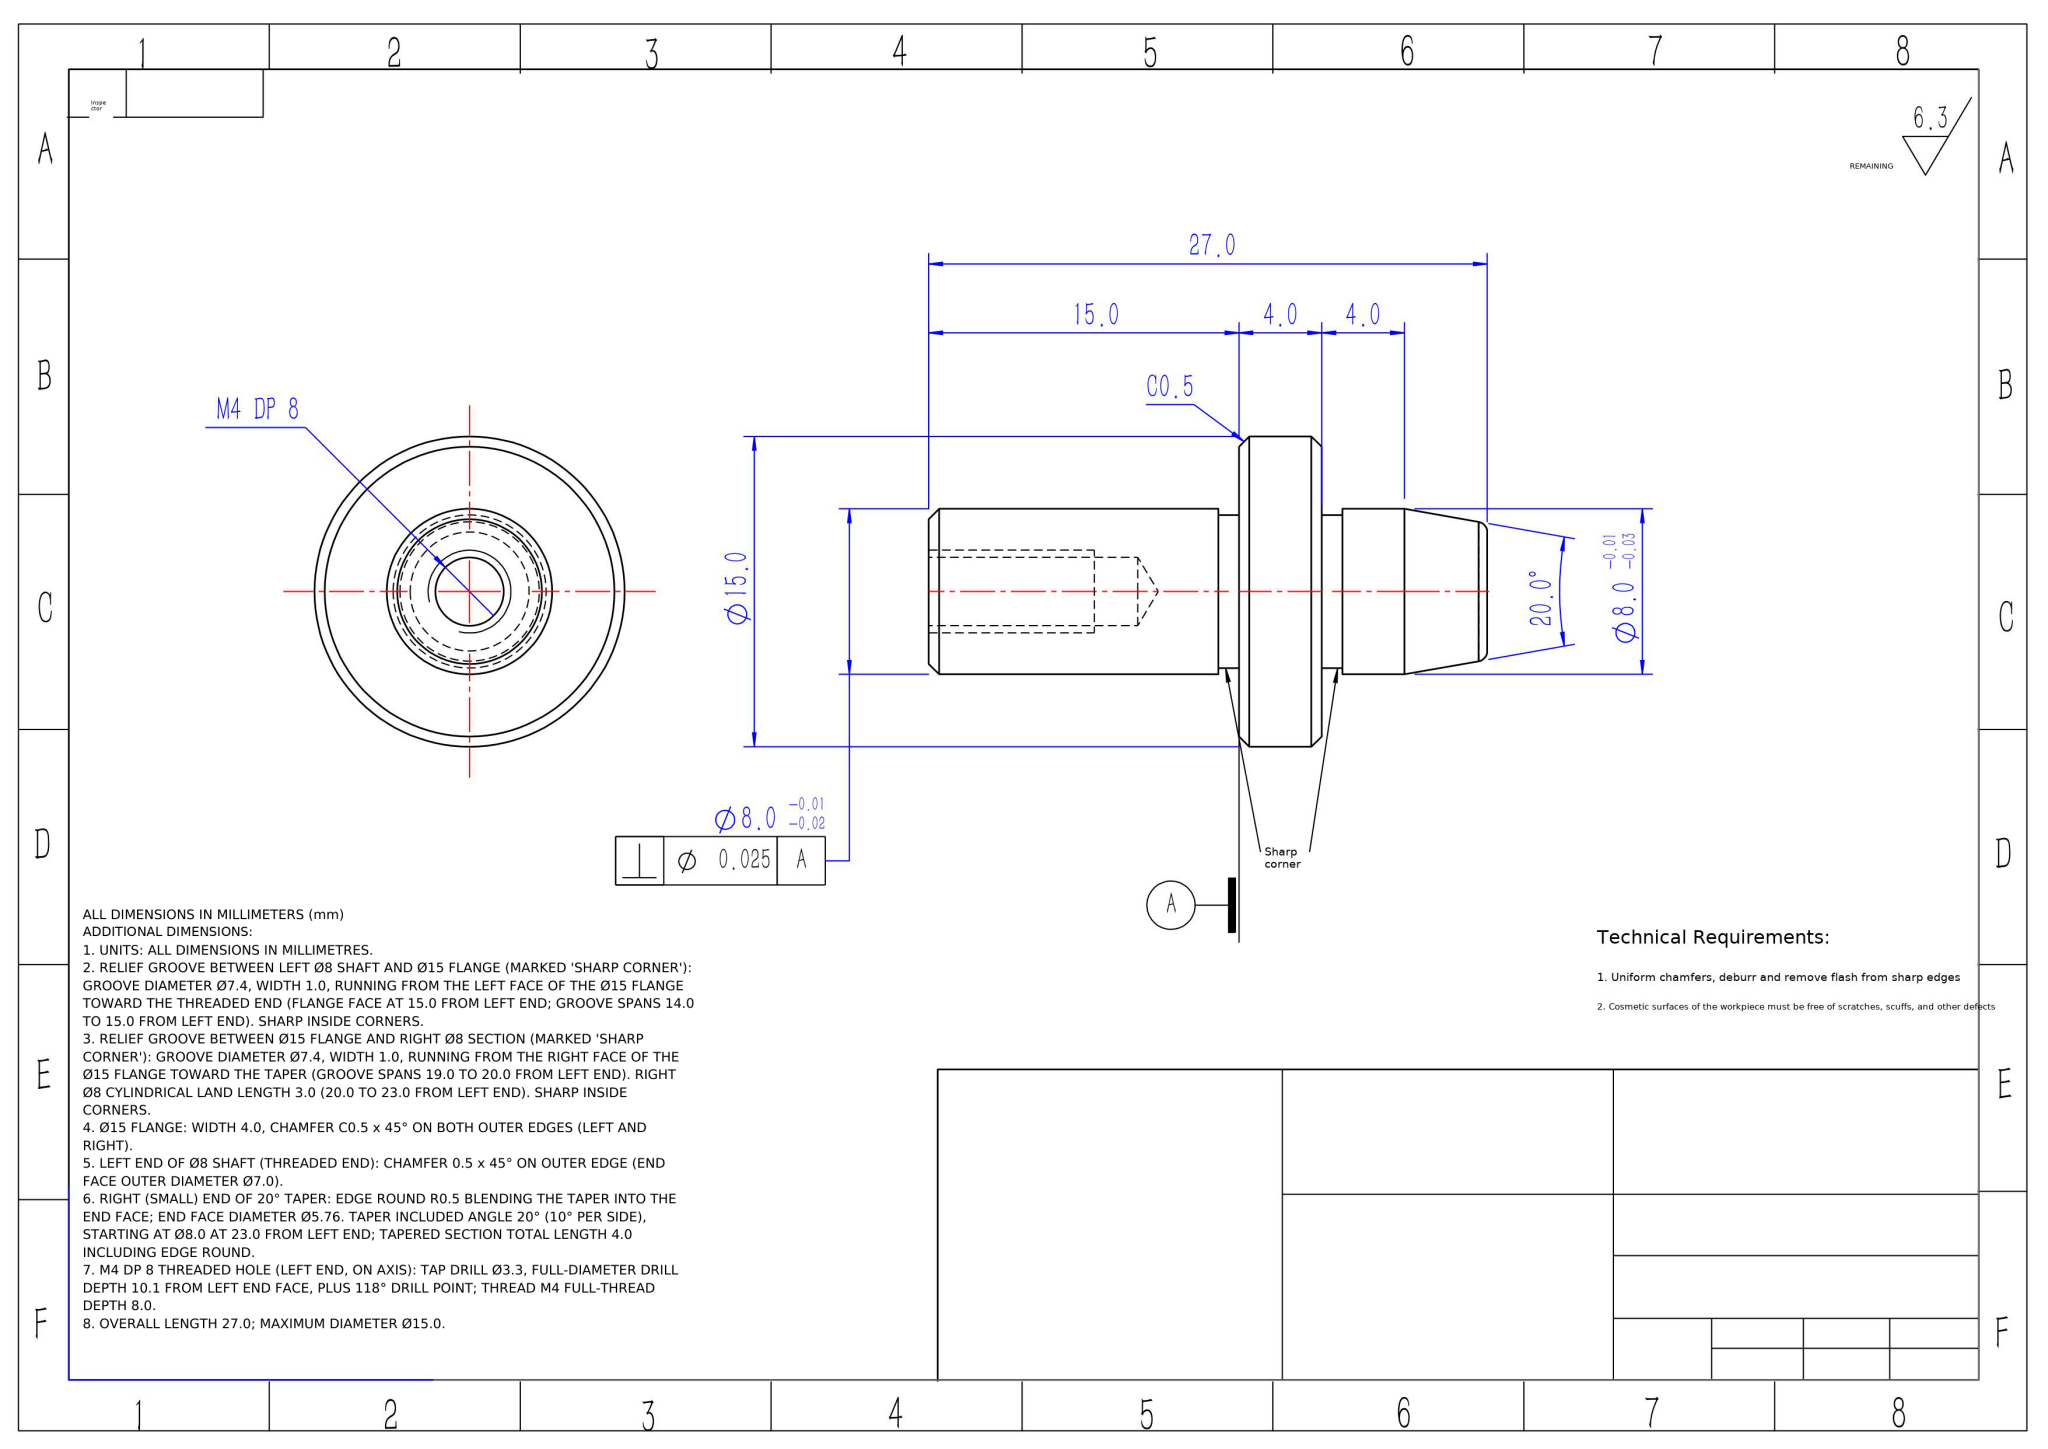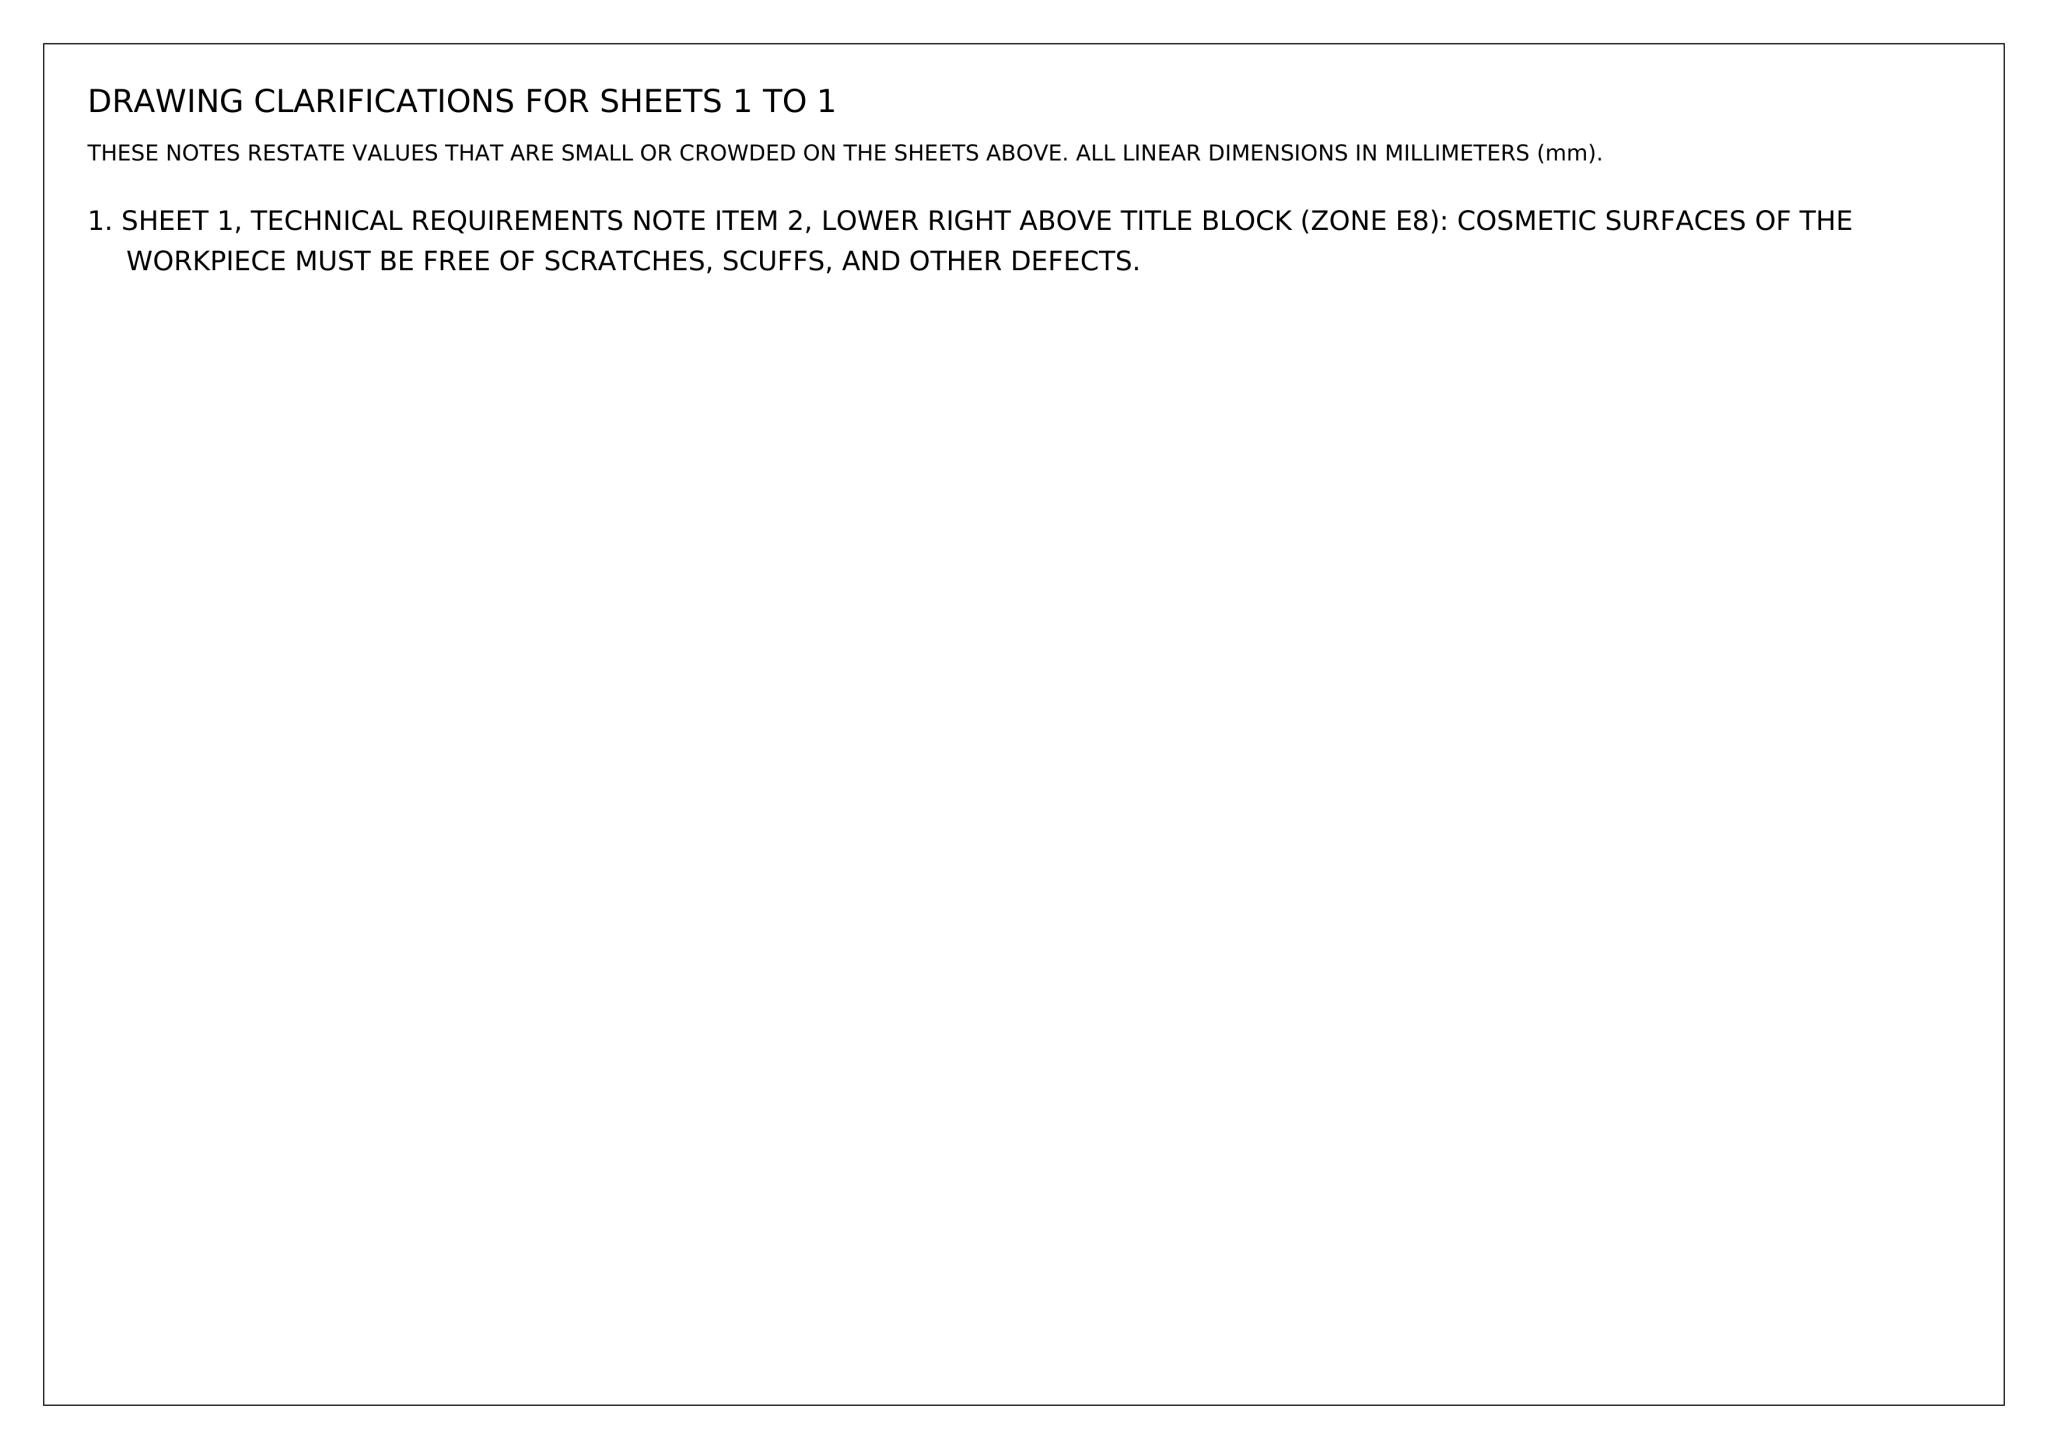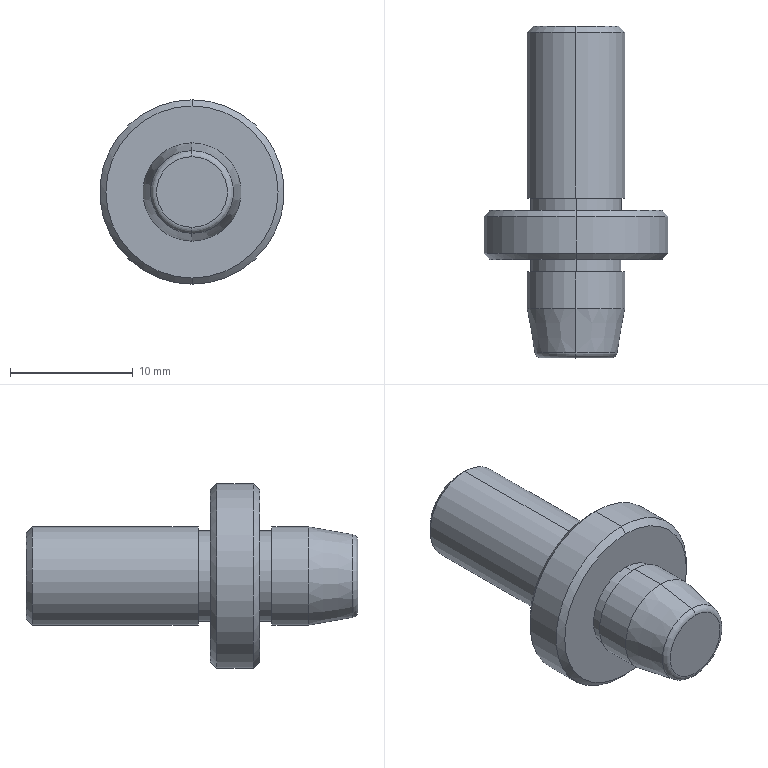Part | NX | mm | Flanged Tubular Connector Pin | 1 solid | 30 faces | box 15 x 27 x 15 mm | volume 1711 mm3 | cylinder 12 | cone 10 | plane 6 | torus 2 | commonest cylinder face diameters 8 x4 7.4 x4 3.3 x2 15 x2